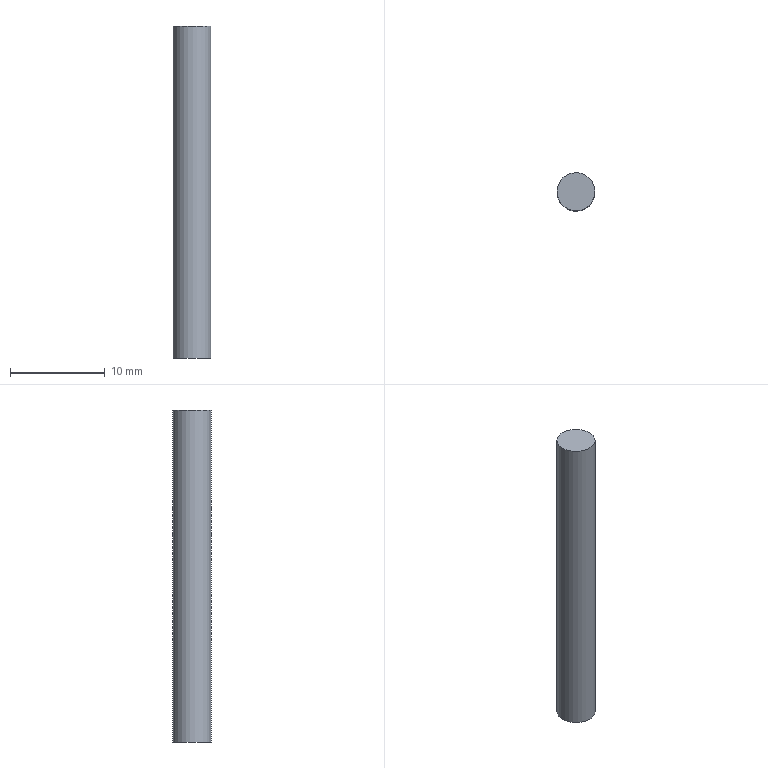Component | NX | STUD_2 | 1 solid | 3 faces | box 4.01 x 4.01 x 35 mm | volume 443 mm3 | plane 2 | cylinder 1 | commonest cylinder face diameters 4.013 x1
STEP:
#1=CARTESIAN_POINT('',(0.,0.,0.));
#2=DIRECTION('',(0.,0.,1.));
#3=DIRECTION('',(1.,0.,0.));
#4=AXIS2_PLACEMENT_3D('',#1,#2,#3);
#5=CARTESIAN_POINT('',(-9.146,10.769,11.5));
#6=VERTEX_POINT('',#5);
#7=CARTESIAN_POINT('',(-11.,10.,11.5));
#8=DIRECTION('',(0.,0.,1.));
#9=DIRECTION('',(0.9237,0.383,0.));
#10=AXIS2_PLACEMENT_3D('',#7,#8,#9);
#11=CIRCLE('',#10,2.007);
#12=CARTESIAN_POINT('',(-11.,10.,11.5));
#13=DIRECTION('',(0.,0.,-1.));
#14=DIRECTION('',(0.9237,0.383,0.));
#15=AXIS2_PLACEMENT_3D('',#12,#13,#14);
#16=PLANE('',#15);
#17=CARTESIAN_POINT('',(2.007,0.));
#18=CARTESIAN_POINT('',(2.007,-3.476));
#19=CARTESIAN_POINT('',(-1.003,-1.738));
#20=CARTESIAN_POINT('',(-4.013,-0.));
#21=CARTESIAN_POINT('',(-1.003,1.738));
#22=CARTESIAN_POINT('',(2.007,3.476));
#23=CARTESIAN_POINT('',(2.007,0.));
#24=(BOUNDED_CURVE()B_SPLINE_CURVE(2,(#17,#18,#19,#20,#21,#22,#23),.UNSPECIFIED.,.T.,.F.)B_SPLINE_CURVE_WITH_KNOTS((1,2,2,2,2,1),(-2.094,0.,2.094,4.189,6.283,8.378),.UNSPECIFIED.)CURVE()GEOMETRIC_REPRESENTATION_ITEM()RATIONAL_B_SPLINE_CURVE((1.,0.5,1.,0.5,1.,0.5,1.))REPRESENTATION_ITEM(''));
#25=(GEOMETRIC_REPRESENTATION_CONTEXT(2)PARAMETRIC_REPRESENTATION_CONTEXT()REPRESENTATION_CONTEXT('',''));
#26=DEFINITIONAL_REPRESENTATION('',(#24),#25);
#27=PCURVE('',#16,#26);
#28=CARTESIAN_POINT('',(-11.,10.,46.5));
#29=DIRECTION('',(0.,0.,-1.));
#30=DIRECTION('',(0.9237,0.383,0.));
#31=AXIS2_PLACEMENT_3D('',#28,#29,#30);
#32=CYLINDRICAL_SURFACE('',#31,2.007);
#33=CARTESIAN_POINT('',(6.283,35.));
#34=DIRECTION('',(-1.,0.));
#35=VECTOR('',#34,1.);
#36=LINE('',#33,#35);
#37=(GEOMETRIC_REPRESENTATION_CONTEXT(2)PARAMETRIC_REPRESENTATION_CONTEXT()REPRESENTATION_CONTEXT('',''));
#38=DEFINITIONAL_REPRESENTATION('',(#36),#37);
#39=PCURVE('',#32,#38);
#40=SURFACE_CURVE('',#11,(#27,#39),.PCURVE_S1.);
#41=EDGE_CURVE('',#6,#6,#40,.T.);
#42=ORIENTED_EDGE('',*,*,#41,.F.);
#43=EDGE_LOOP('',(#42));
#44=FACE_BOUND('',#43,.T.);
#45=ADVANCED_FACE('',(#44),#16,.T.);
#46=CARTESIAN_POINT('',(-9.146,10.769,46.5));
#47=VERTEX_POINT('',#46);
#48=CARTESIAN_POINT('',(-11.,10.,46.5));
#49=DIRECTION('',(0.,0.,-1.));
#50=DIRECTION('',(0.9237,0.383,0.));
#51=AXIS2_PLACEMENT_3D('',#48,#49,#50);
#52=CIRCLE('',#51,2.007);
#53=CARTESIAN_POINT('',(-11.,10.,46.5));
#54=DIRECTION('',(0.,0.,1.));
#55=DIRECTION('',(-0.9237,-0.383,0.));
#56=AXIS2_PLACEMENT_3D('',#53,#54,#55);
#57=PLANE('',#56);
#58=CARTESIAN_POINT('',(-2.007,0.));
#59=CARTESIAN_POINT('',(-2.007,3.476));
#60=CARTESIAN_POINT('',(1.003,1.738));
#61=CARTESIAN_POINT('',(4.013,0.));
#62=CARTESIAN_POINT('',(1.003,-1.738));
#63=CARTESIAN_POINT('',(-2.007,-3.476));
#64=CARTESIAN_POINT('',(-2.007,0.));
#65=(BOUNDED_CURVE()B_SPLINE_CURVE(2,(#58,#59,#60,#61,#62,#63,#64),.UNSPECIFIED.,.T.,.F.)B_SPLINE_CURVE_WITH_KNOTS((1,2,2,2,2,1),(-2.094,0.,2.094,4.189,6.283,8.378),.UNSPECIFIED.)CURVE()GEOMETRIC_REPRESENTATION_ITEM()RATIONAL_B_SPLINE_CURVE((1.,0.5,1.,0.5,1.,0.5,1.))REPRESENTATION_ITEM(''));
#66=(GEOMETRIC_REPRESENTATION_CONTEXT(2)PARAMETRIC_REPRESENTATION_CONTEXT()REPRESENTATION_CONTEXT('',''));
#67=DEFINITIONAL_REPRESENTATION('',(#65),#66);
#68=PCURVE('',#57,#67);
#69=CARTESIAN_POINT('',(0.,0.));
#70=DIRECTION('',(1.,0.));
#71=VECTOR('',#70,1.);
#72=LINE('',#69,#71);
#73=(GEOMETRIC_REPRESENTATION_CONTEXT(2)PARAMETRIC_REPRESENTATION_CONTEXT()REPRESENTATION_CONTEXT('',''));
#74=DEFINITIONAL_REPRESENTATION('',(#72),#73);
#75=PCURVE('',#32,#74);
#76=SURFACE_CURVE('',#52,(#68,#75),.PCURVE_S1.);
#77=EDGE_CURVE('',#47,#47,#76,.T.);
#78=ORIENTED_EDGE('',*,*,#77,.F.);
#79=EDGE_LOOP('',(#78));
#80=FACE_BOUND('',#79,.T.);
#81=ADVANCED_FACE('',(#80),#57,.T.);
#82=ORIENTED_EDGE('',*,*,#41,.T.);
#83=CARTESIAN_POINT('',(-9.146,10.769,46.5));
#84=CARTESIAN_POINT('',(-9.146,10.769,11.5));
#85=B_SPLINE_CURVE_WITH_KNOTS('',1,(#83,#84),.UNSPECIFIED.,.F.,.F.,(2,2),(0.,35.),.PIECEWISE_BEZIER_KNOTS.);
#86=CARTESIAN_POINT('',(0.,0.));
#87=DIRECTION('',(0.,1.));
#88=VECTOR('',#87,1.);
#89=LINE('',#86,#88);
#90=(GEOMETRIC_REPRESENTATION_CONTEXT(2)PARAMETRIC_REPRESENTATION_CONTEXT()REPRESENTATION_CONTEXT('',''));
#91=DEFINITIONAL_REPRESENTATION('',(#89),#90);
#92=PCURVE('',#32,#91);
#93=CARTESIAN_POINT('',(6.283,0.));
#94=DIRECTION('',(0.,1.));
#95=VECTOR('',#94,1.);
#96=LINE('',#93,#95);
#97=(GEOMETRIC_REPRESENTATION_CONTEXT(2)PARAMETRIC_REPRESENTATION_CONTEXT()REPRESENTATION_CONTEXT('',''));
#98=DEFINITIONAL_REPRESENTATION('',(#96),#97);
#99=PCURVE('',#32,#98);
#100=SEAM_CURVE('',#85,(#92,#99),.PCURVE_S1.);
#101=EDGE_CURVE('',#47,#6,#100,.T.);
#102=ORIENTED_EDGE('',*,*,#101,.F.);
#103=ORIENTED_EDGE('',*,*,#77,.T.);
#104=ORIENTED_EDGE('',*,*,#101,.T.);
#105=EDGE_LOOP('',(#82,#102,#103,#104));
#106=FACE_BOUND('',#105,.T.);
#107=ADVANCED_FACE('',(#106),#32,.T.);
#108=CLOSED_SHELL('',(#45,#81,#107));
#109=MANIFOLD_SOLID_BREP('',#108);
#110=(LENGTH_UNIT()NAMED_UNIT(*)SI_UNIT(.MILLI.,.METRE.));
#111=UNCERTAINTY_MEASURE_WITH_UNIT(LENGTH_MEASURE(0.00001),#110,'','');
#112=(NAMED_UNIT(*)PLANE_ANGLE_UNIT()SI_UNIT($,.RADIAN.));
#113=(NAMED_UNIT(*)SI_UNIT($,.STERADIAN.)SOLID_ANGLE_UNIT());
#114=(GEOMETRIC_REPRESENTATION_CONTEXT(3)GLOBAL_UNCERTAINTY_ASSIGNED_CONTEXT((#111))GLOBAL_UNIT_ASSIGNED_CONTEXT((#110,#112,#113))REPRESENTATION_CONTEXT('',''));
#115=ADVANCED_BREP_SHAPE_REPRESENTATION('',(#4,#109),#114);